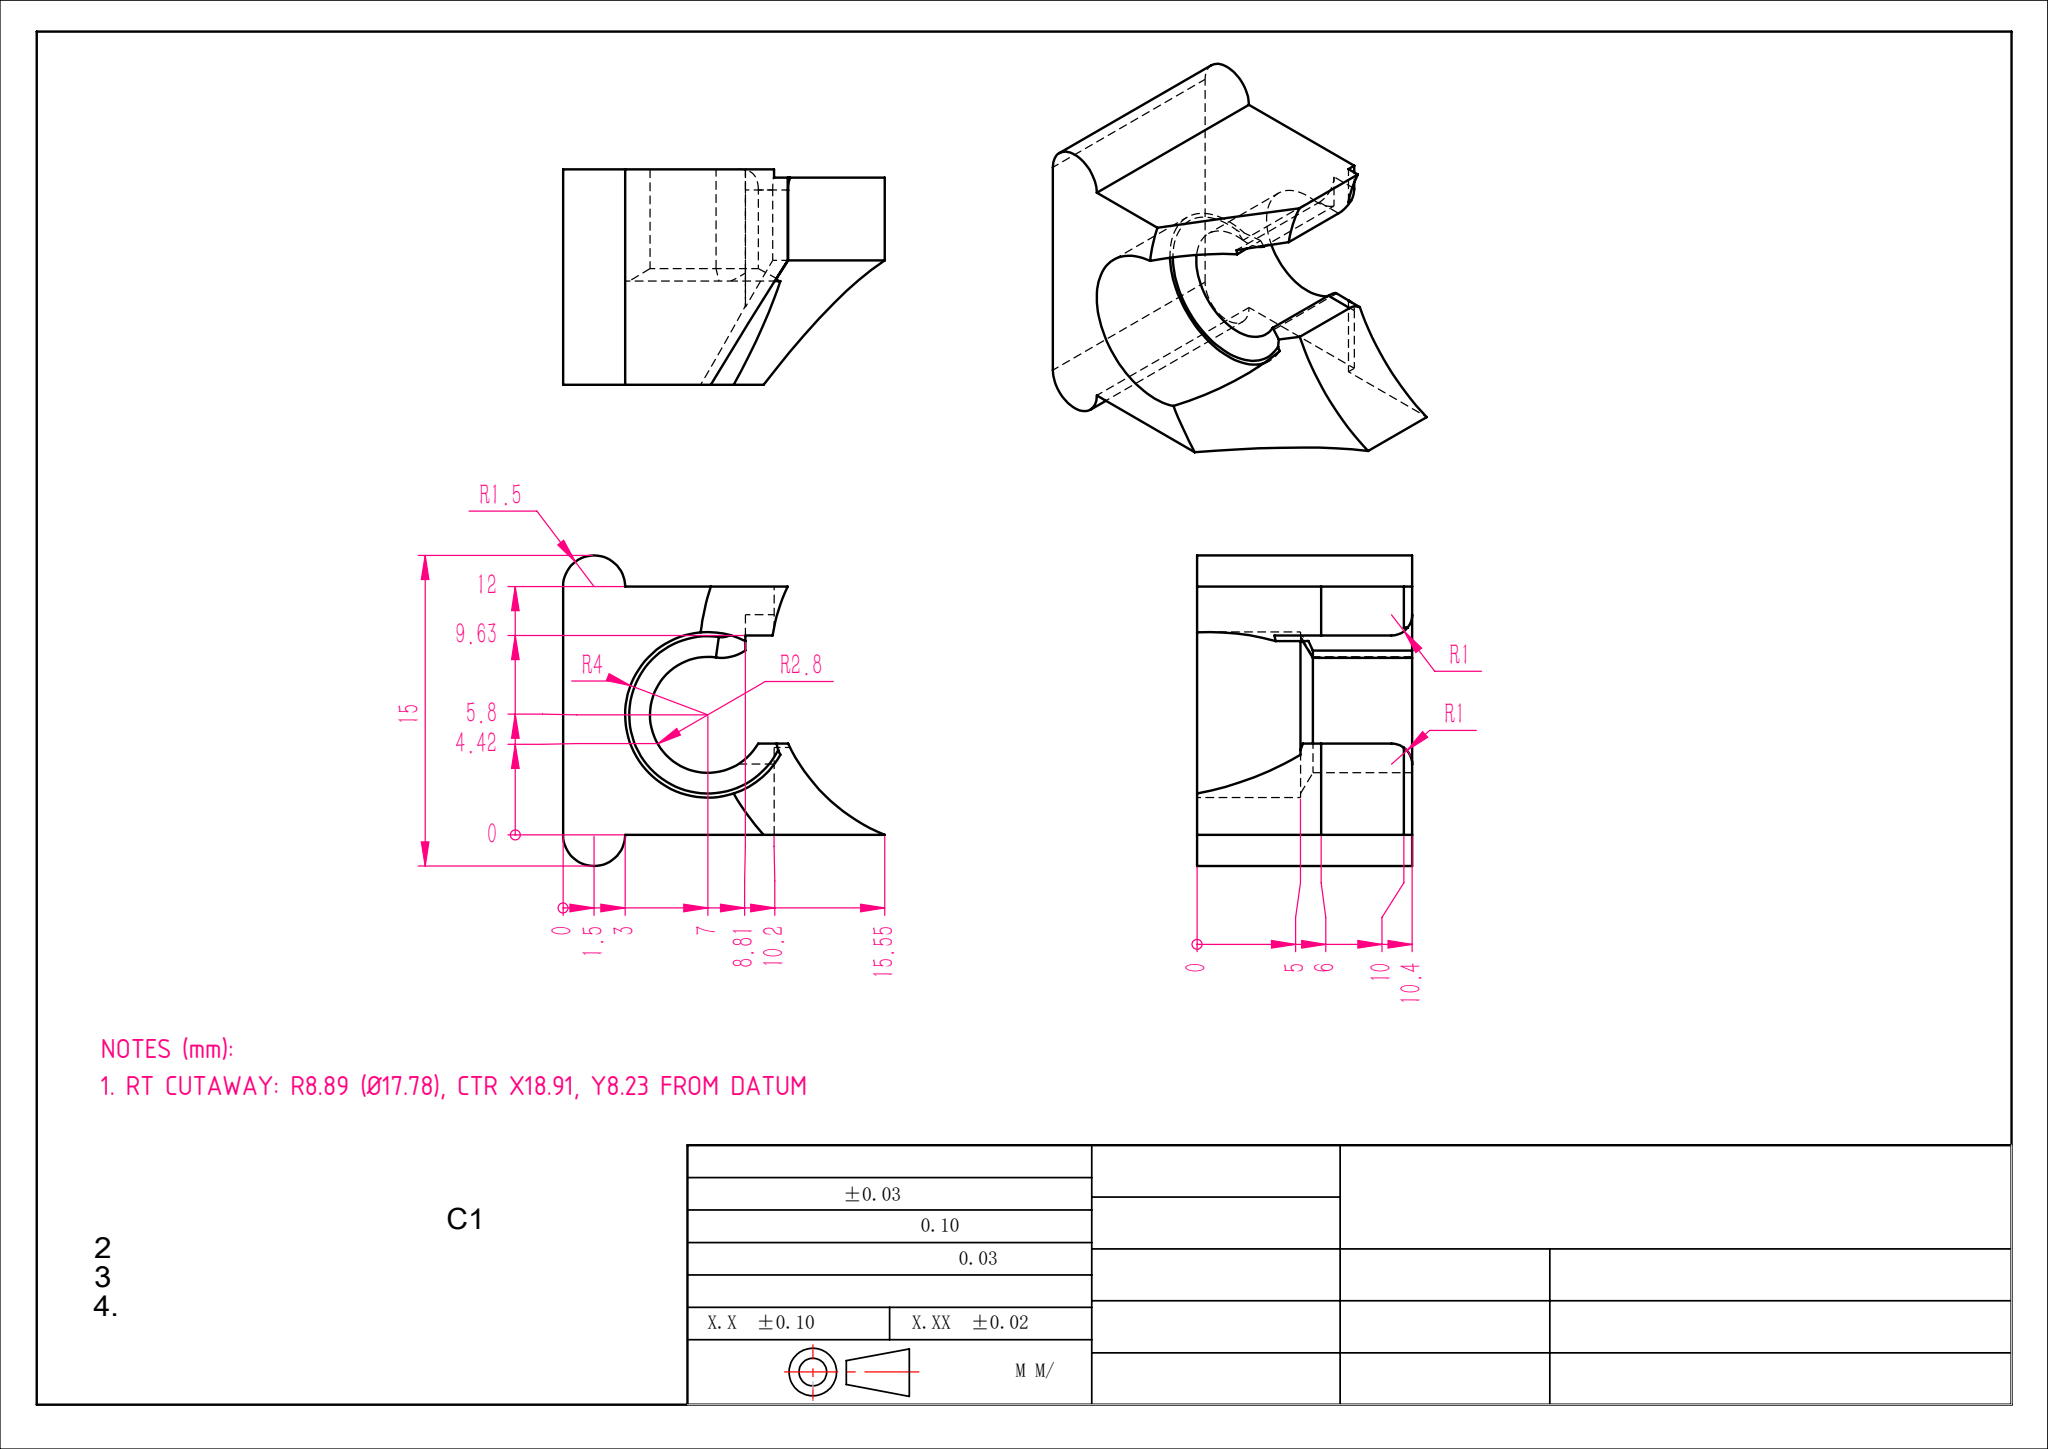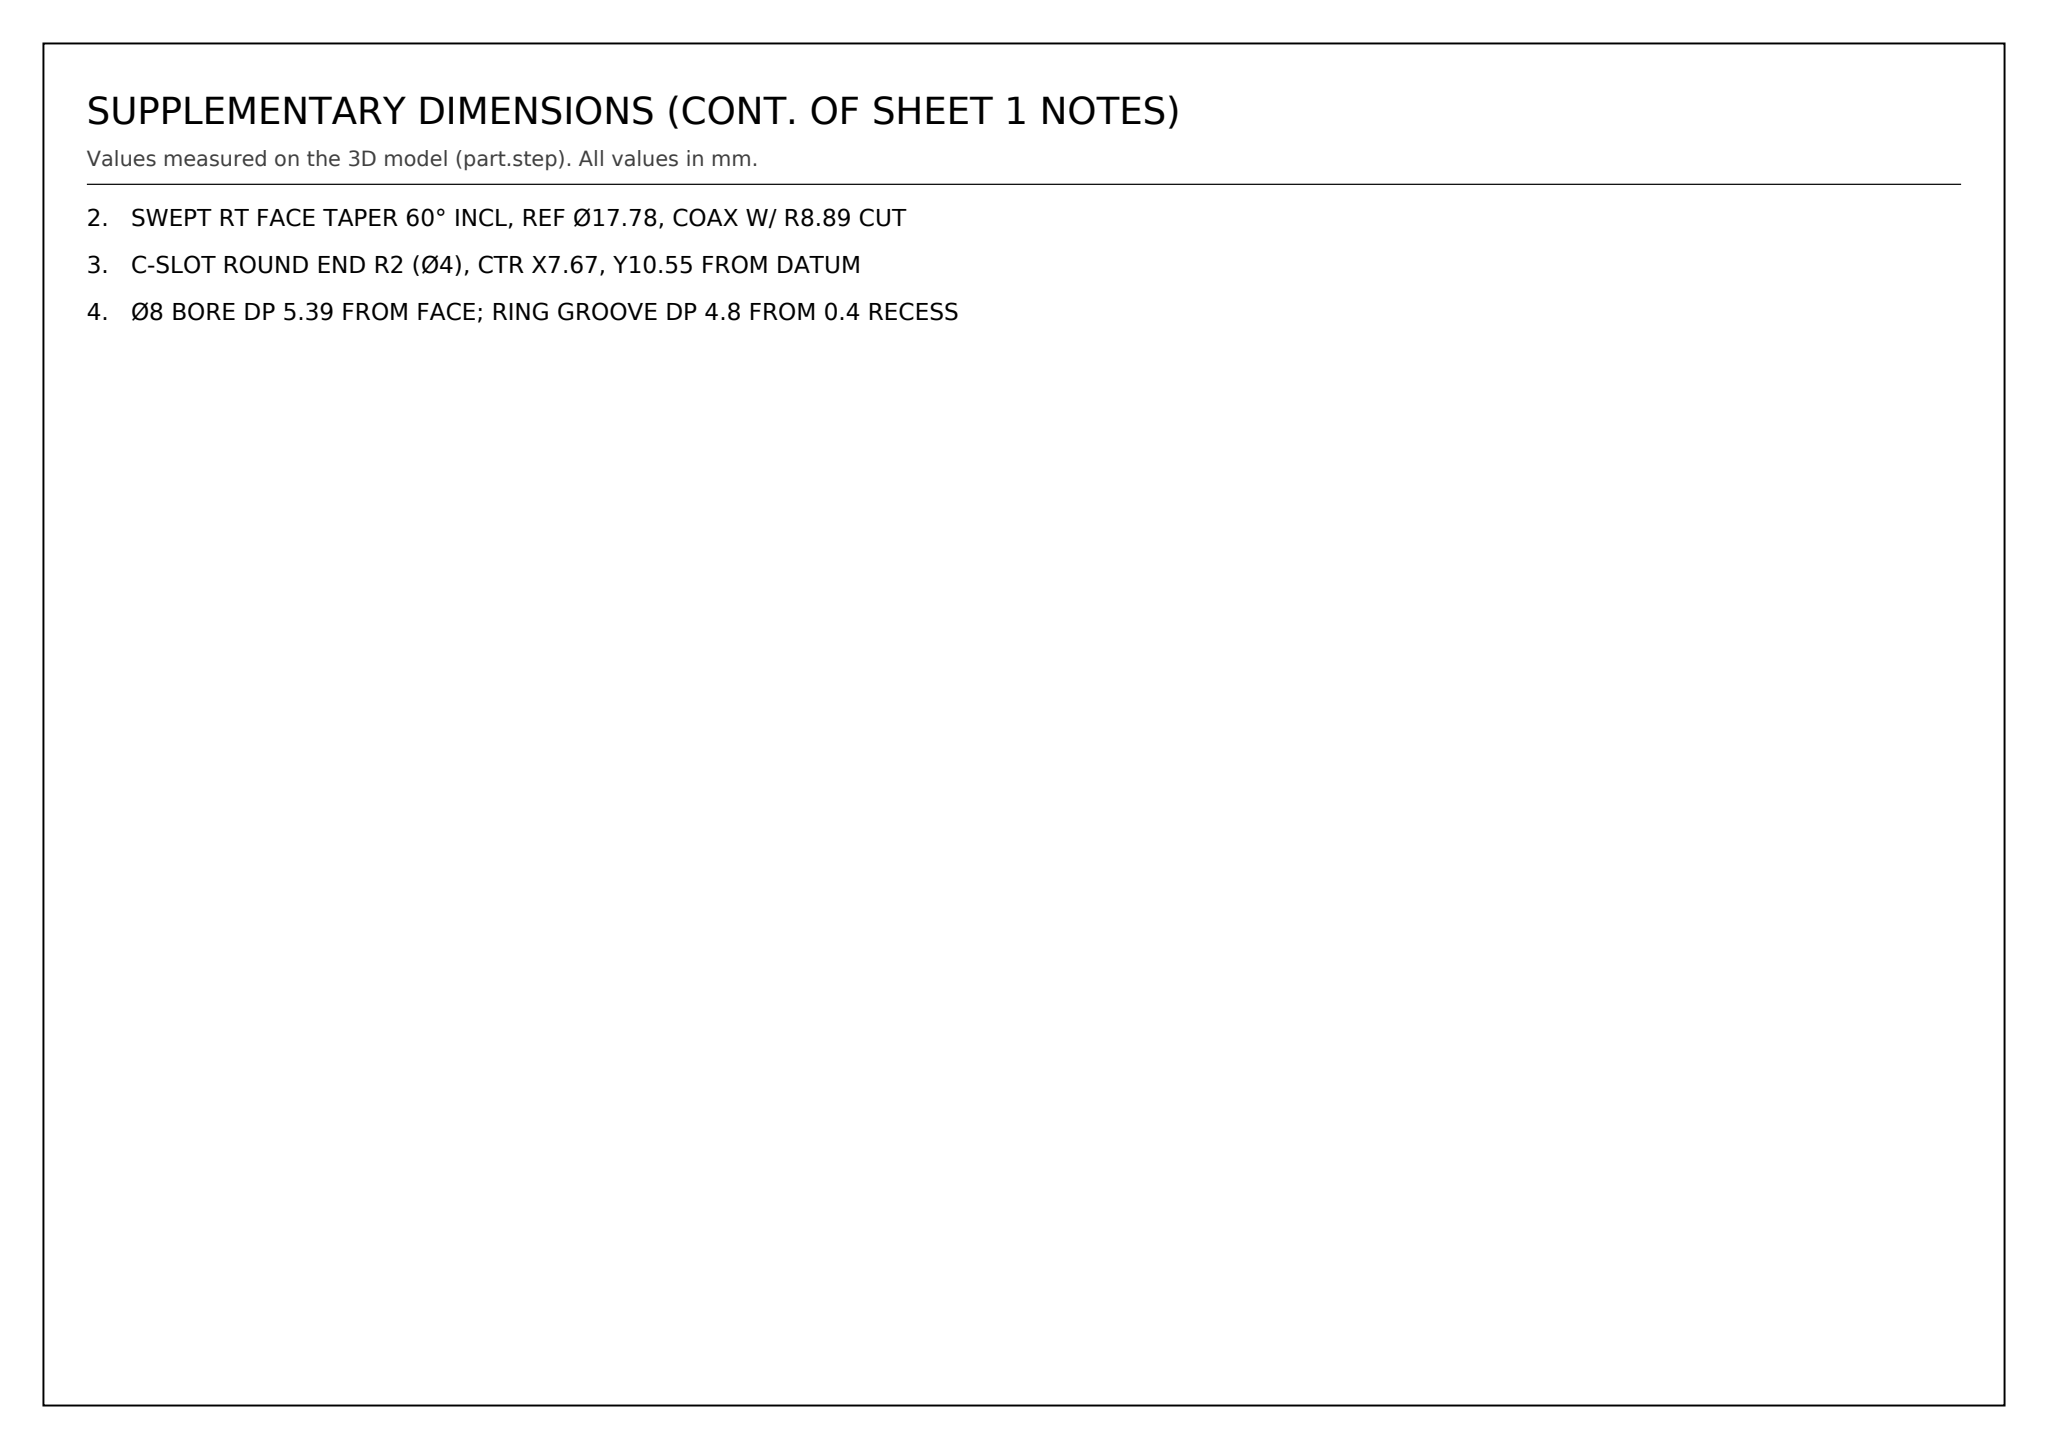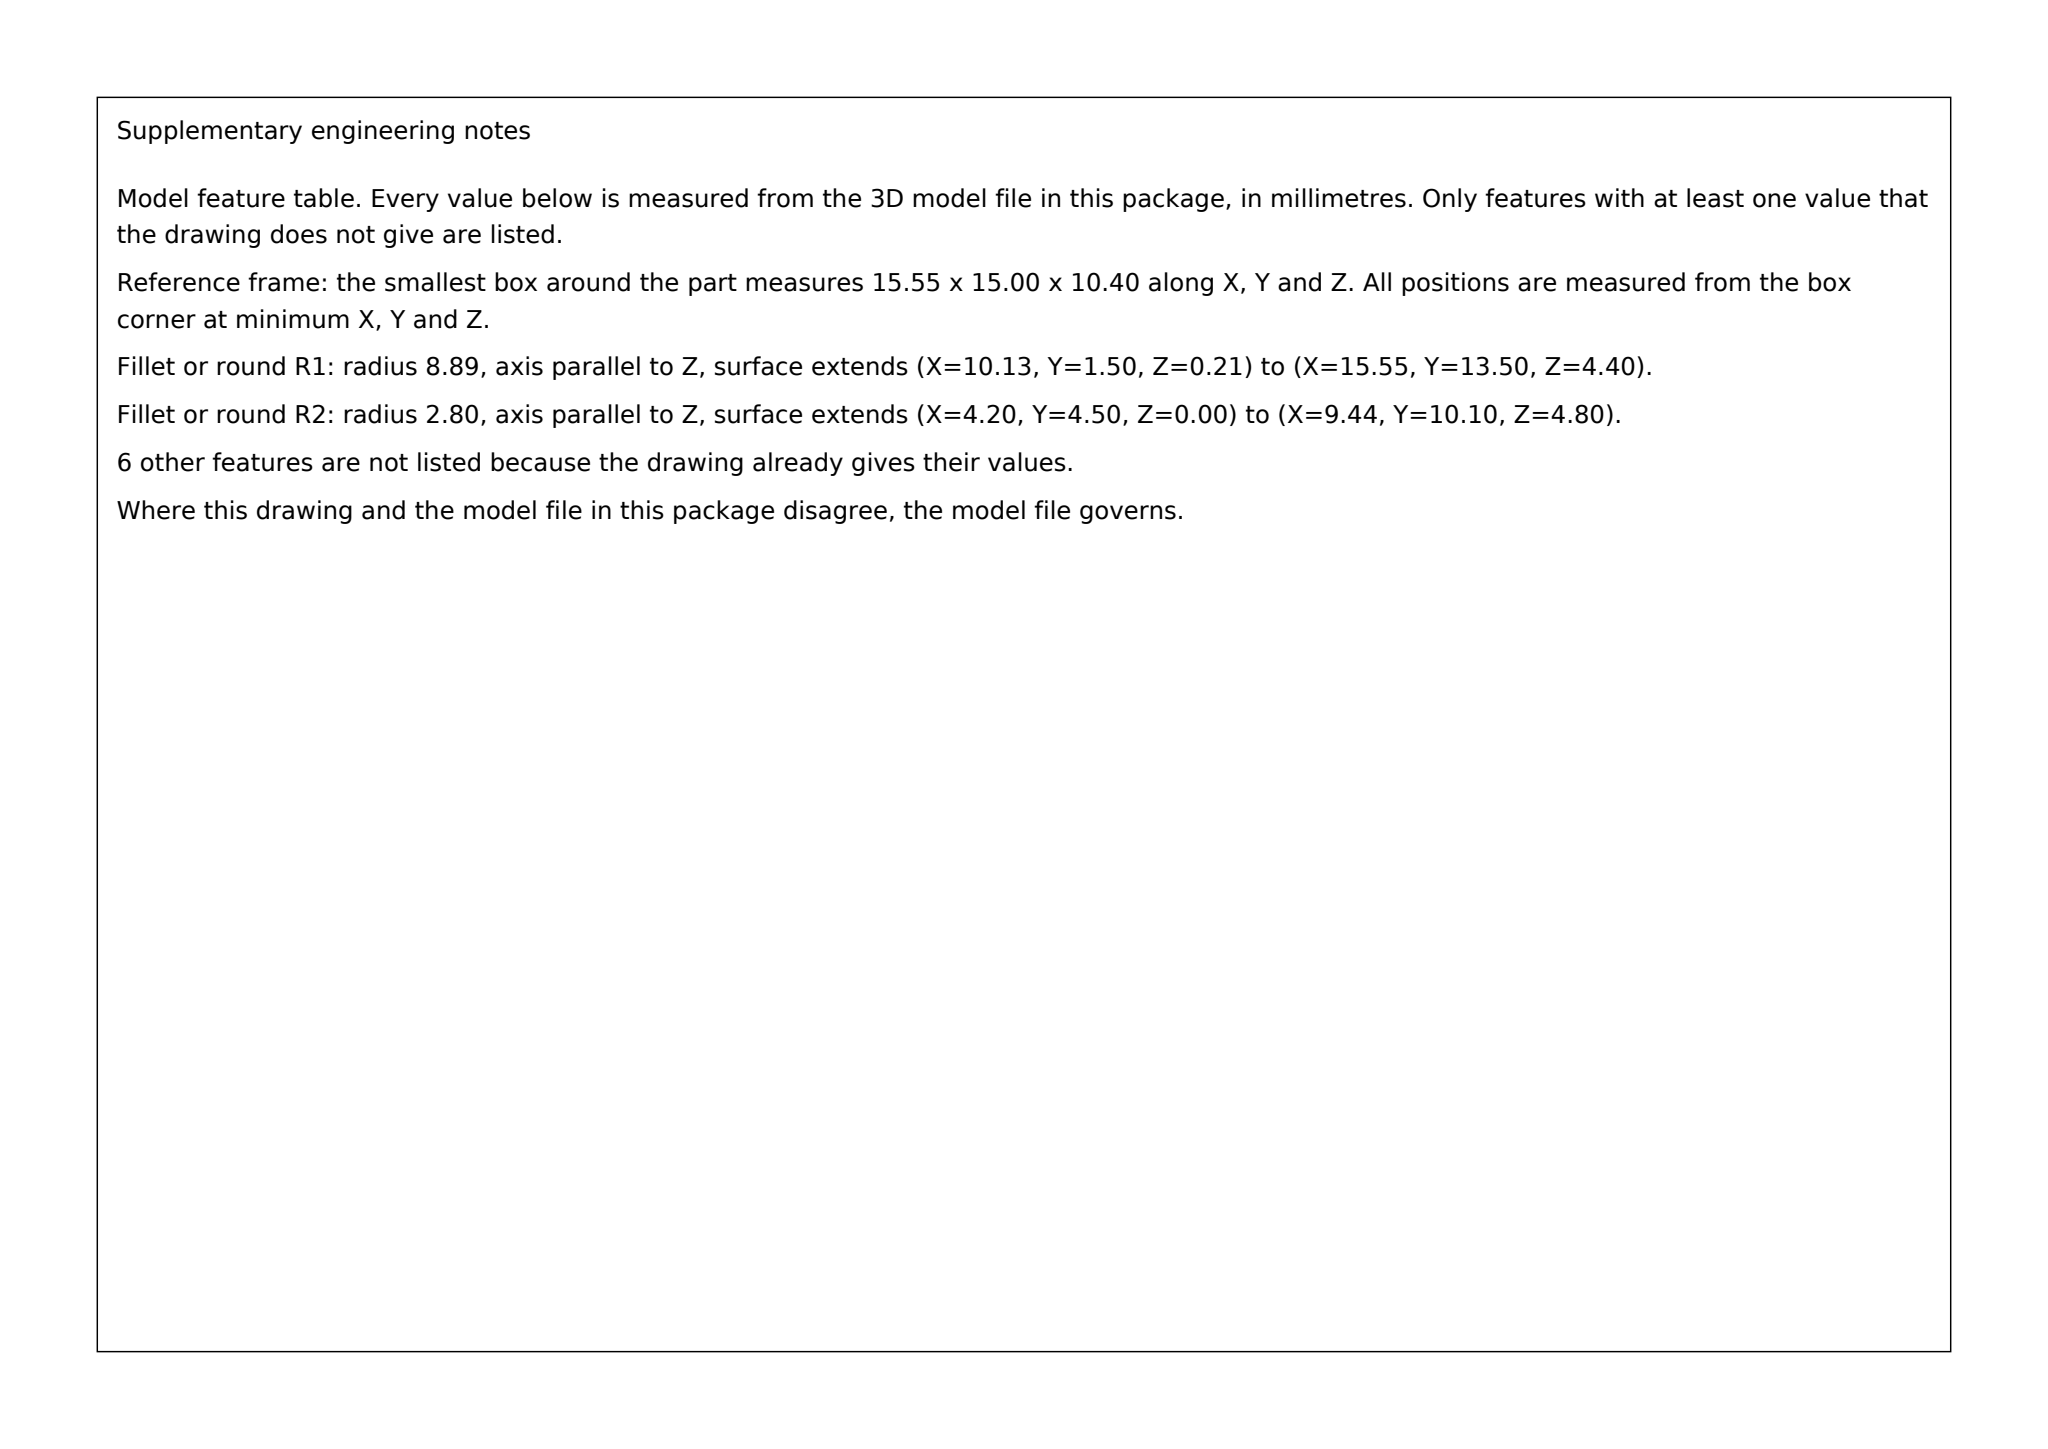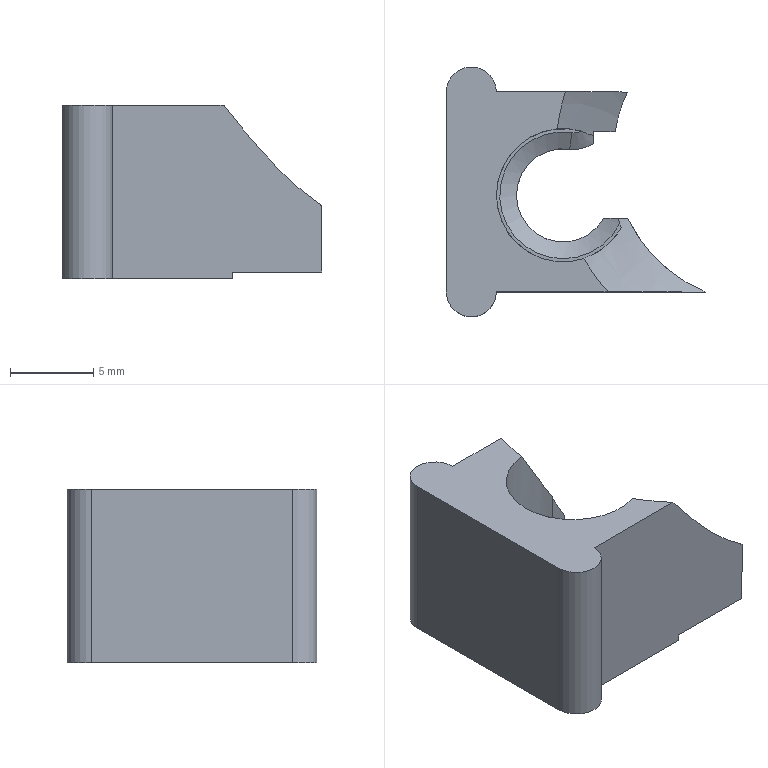Part | SolidWorks | mm | 1 solid | 27 faces | box 15.55 x 15 x 10.4 mm | volume 974 mm3 | plane 13 | cylinder 10 | cone 4 | commonest cylinder face diameters 5.6 x2 3 x2 17.784 x2 2 x2 4 x1 8 x1
Drawing notes:
RT CUTAWAY: R8.89 (Ø17.78), CTR X18.91, Y8.23 FROM DATUM | from the solid: cylinder dia 17.784, axis z, pos (18.91, 11.44); drawing Y datum = bbox y 3.21, so Y = 11.44-3.21 = 8.23; leftmost pt x=10.02 and bottom intersect x=15.54 match dims 10.2/15.55
SWEPT RT FACE TAPER 60° INCL, REF Ø17.78, COAX W/ R8.89 CUT | from the solid: cones[included_angle,ref_dia] = [60.0, 17.784] x2, same axis as Ø17.784 cyl at (18.91, 11.44)
C-SLOT ROUND END R2 (Ø4), CTR X7.67, Y10.55 FROM DATUM | from the solid: cylinder dia 4.0, axis z, pos (7.67, 13.76), len 4.8; Y = 13.76-3.21 = 10.55 in drawing datum
Ø8 BORE DP 5.39 FROM FACE; RING GROOVE DP 4.8 FROM 0.4 RECESS | from the solid: cyl dia 8 len 5.39; cyl dia 5.6 (x2) and dia 4 len 4.8; z planes 0, 0.4 (x2), 5.4, 10.4 give 0.4 recessed ledge